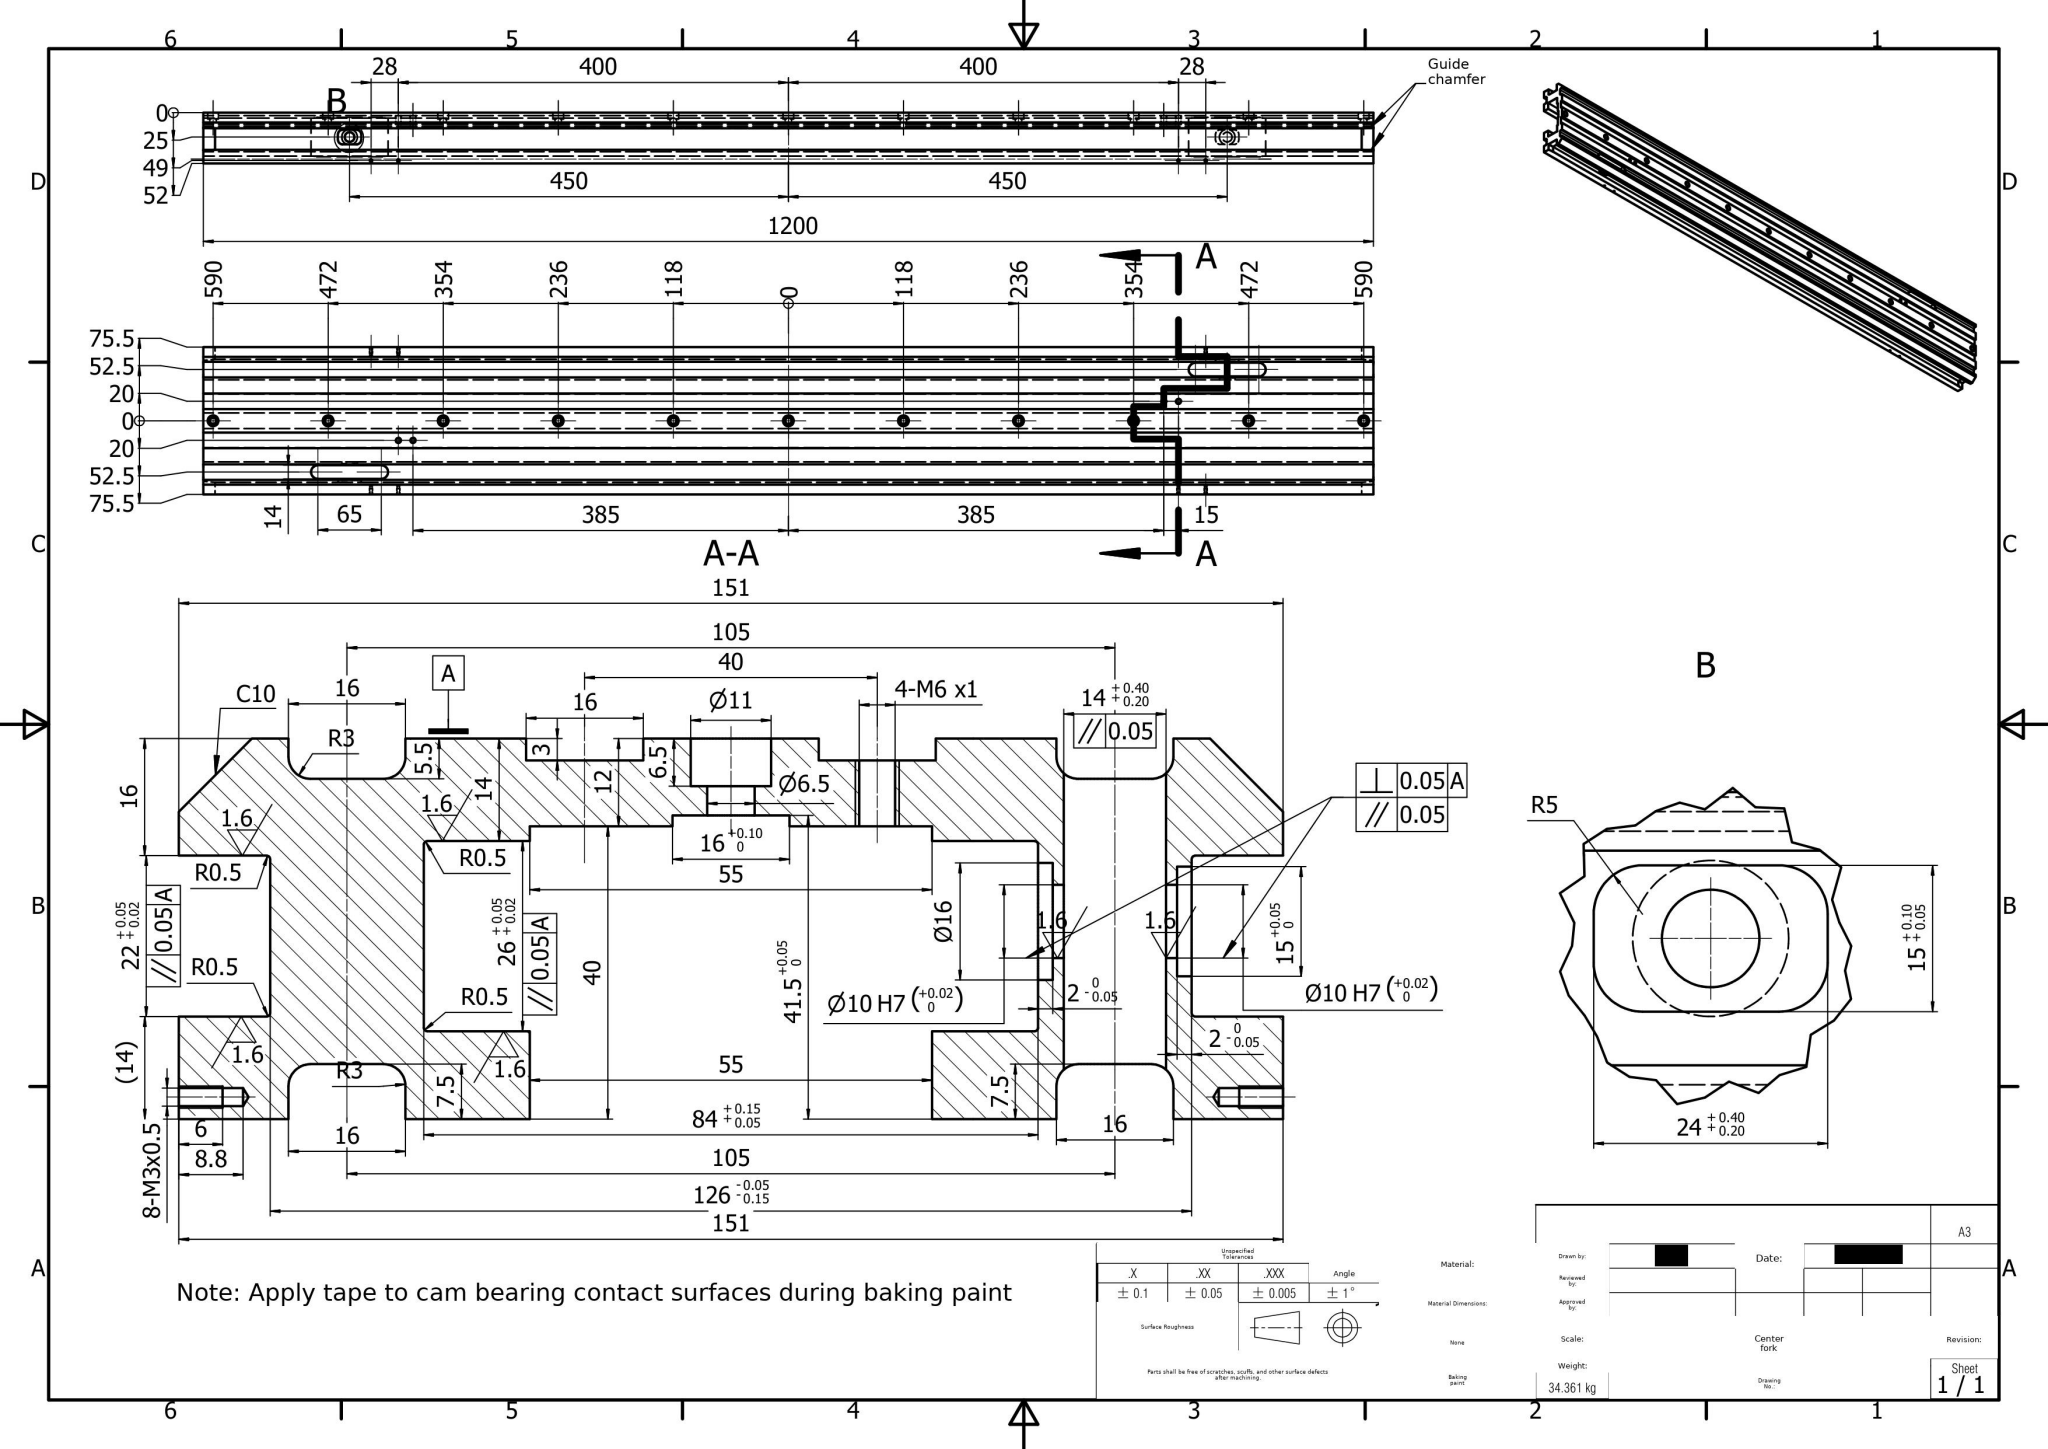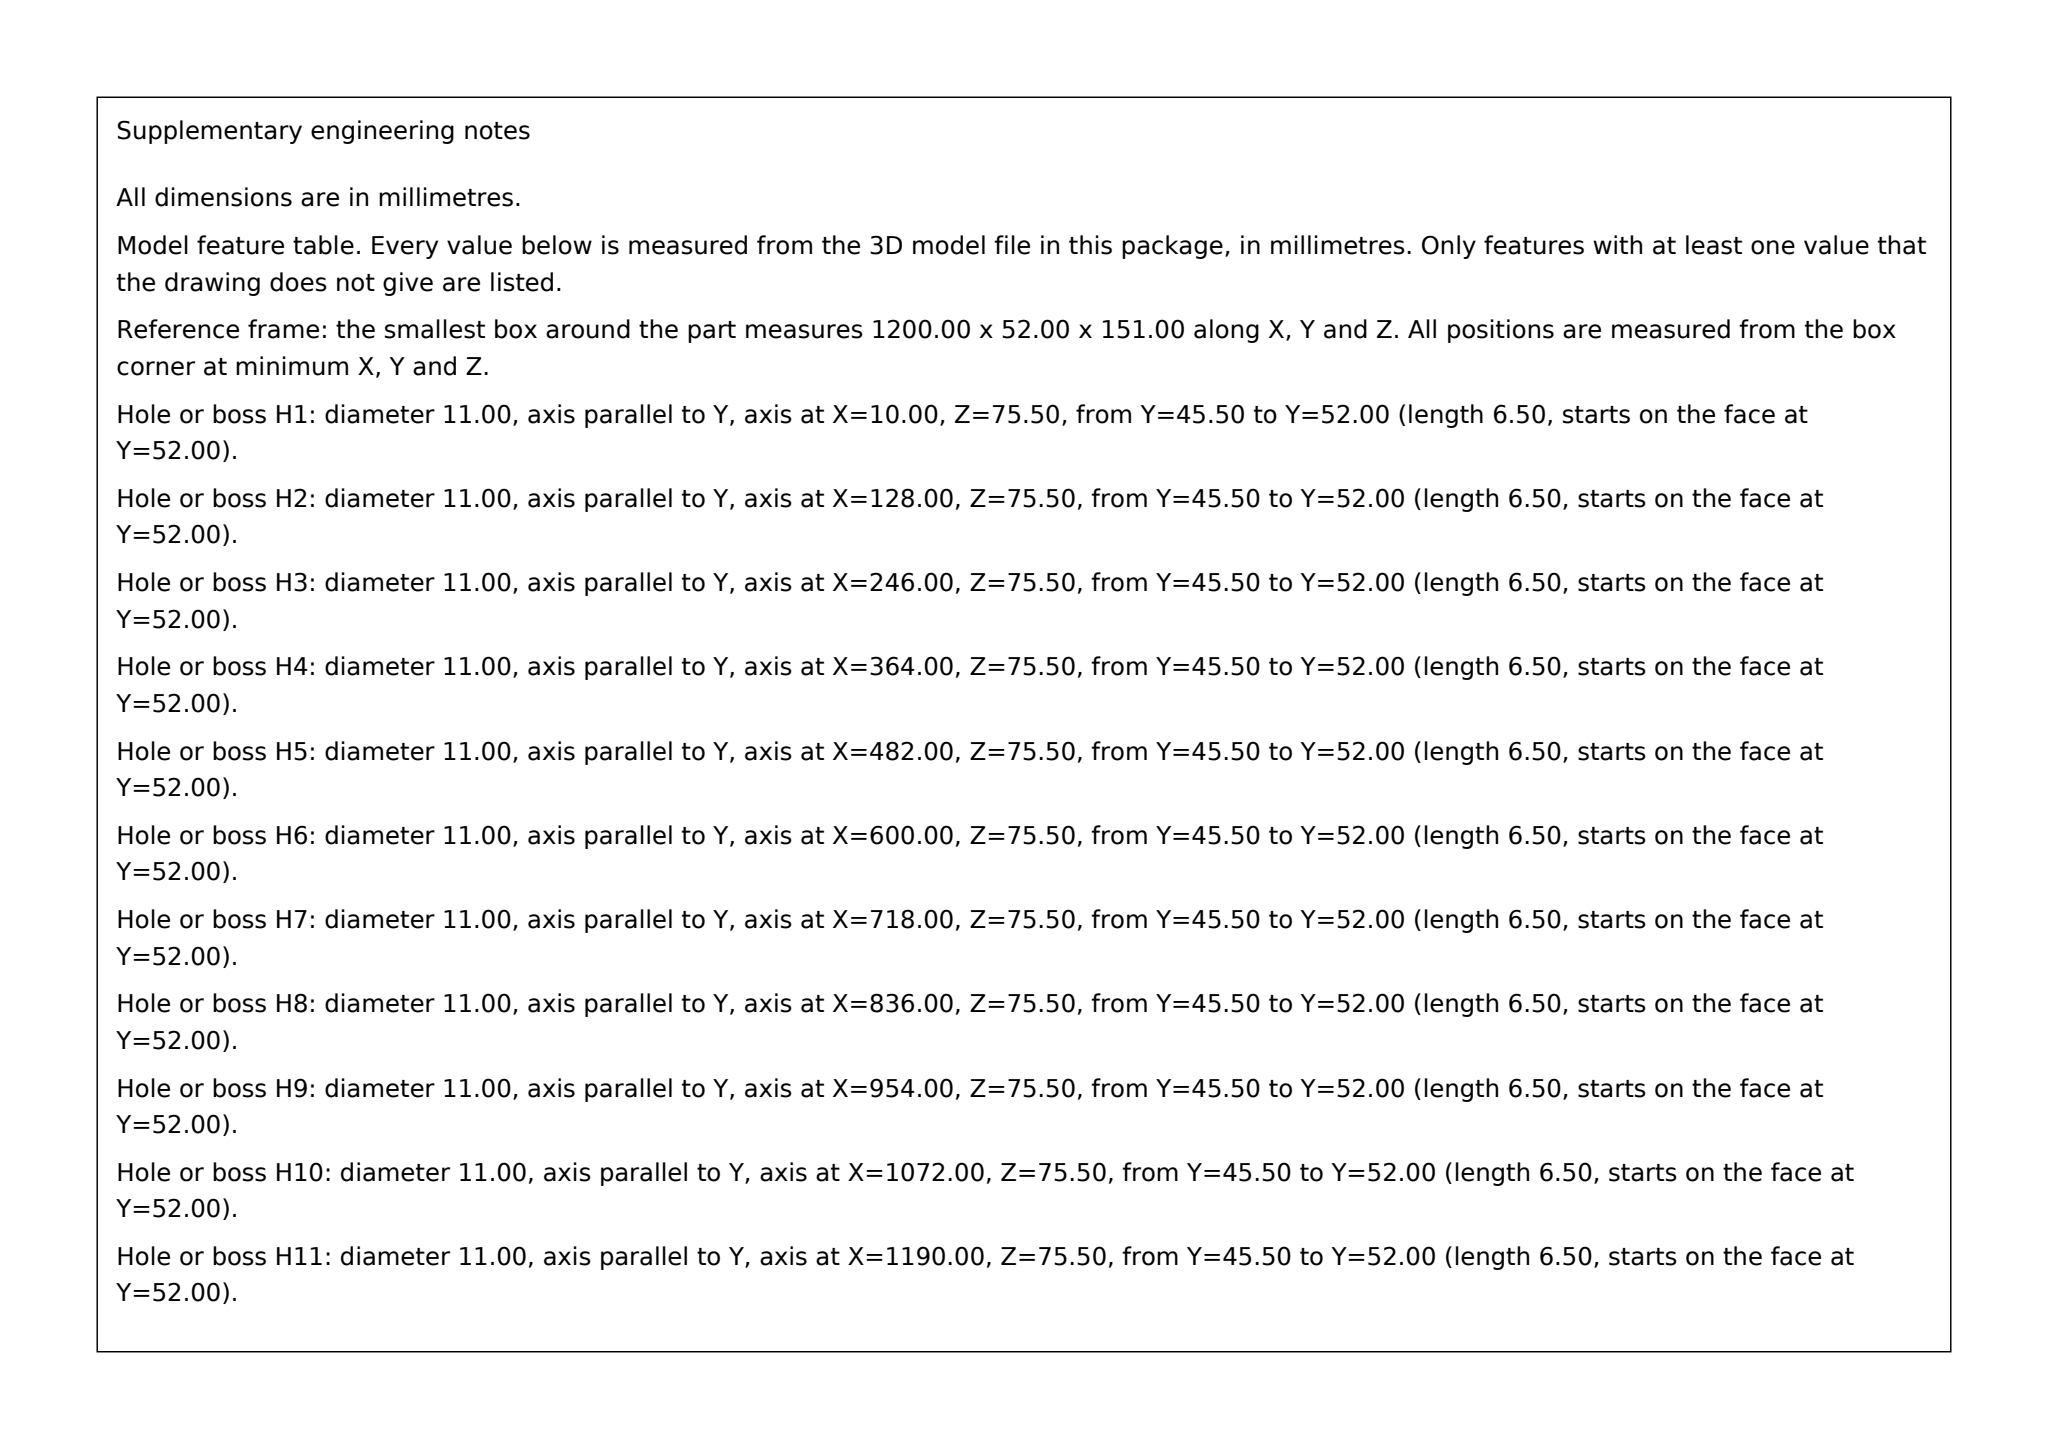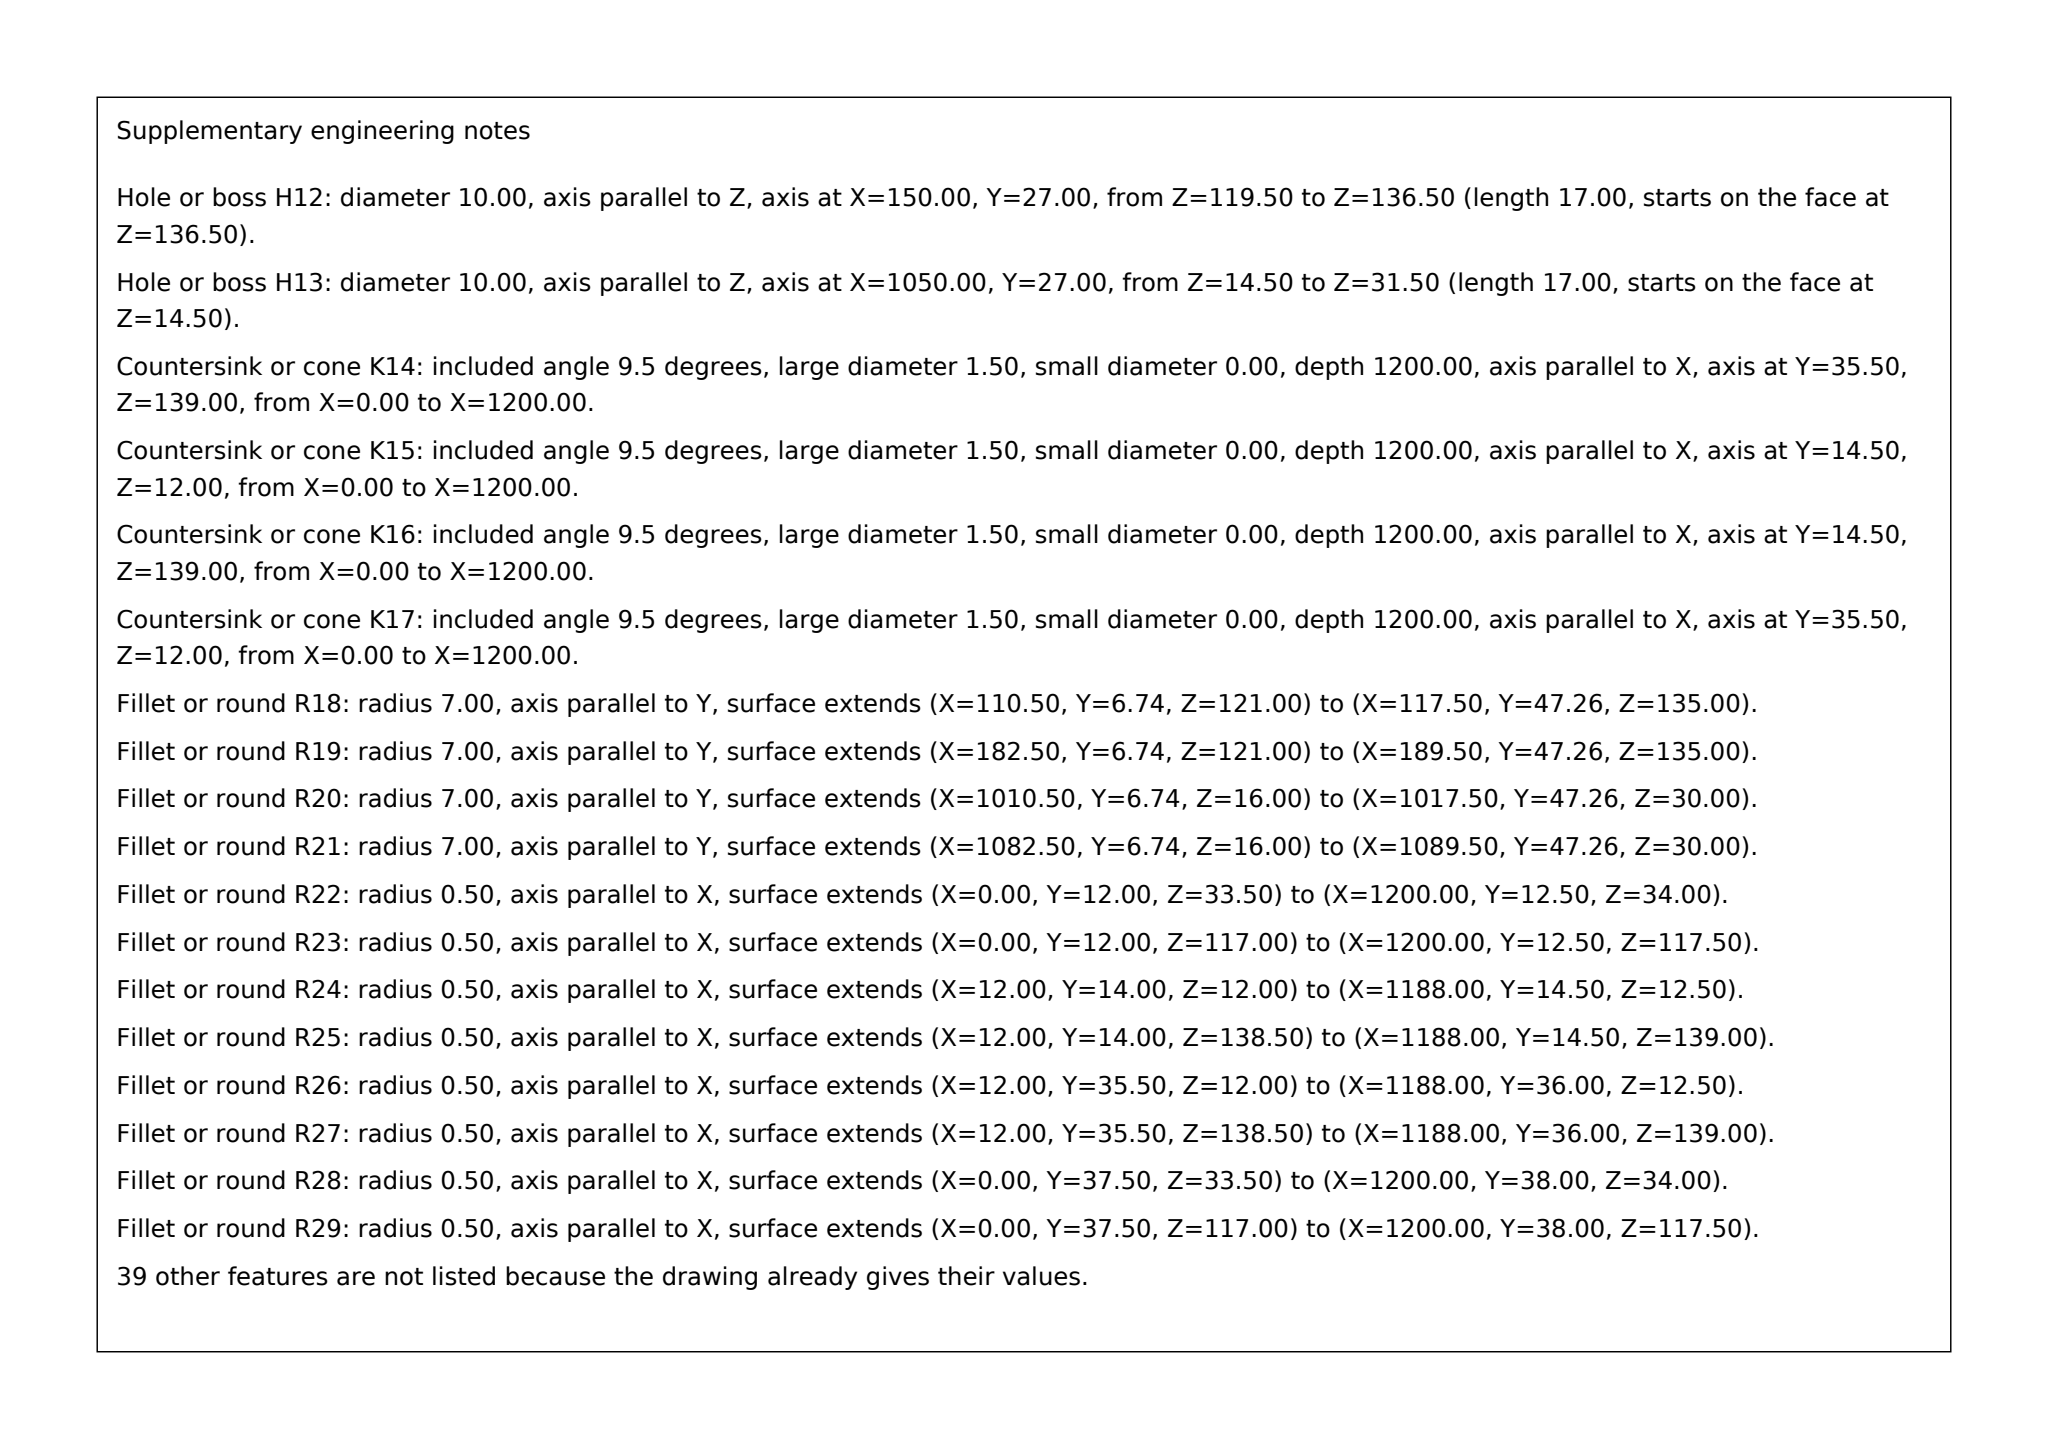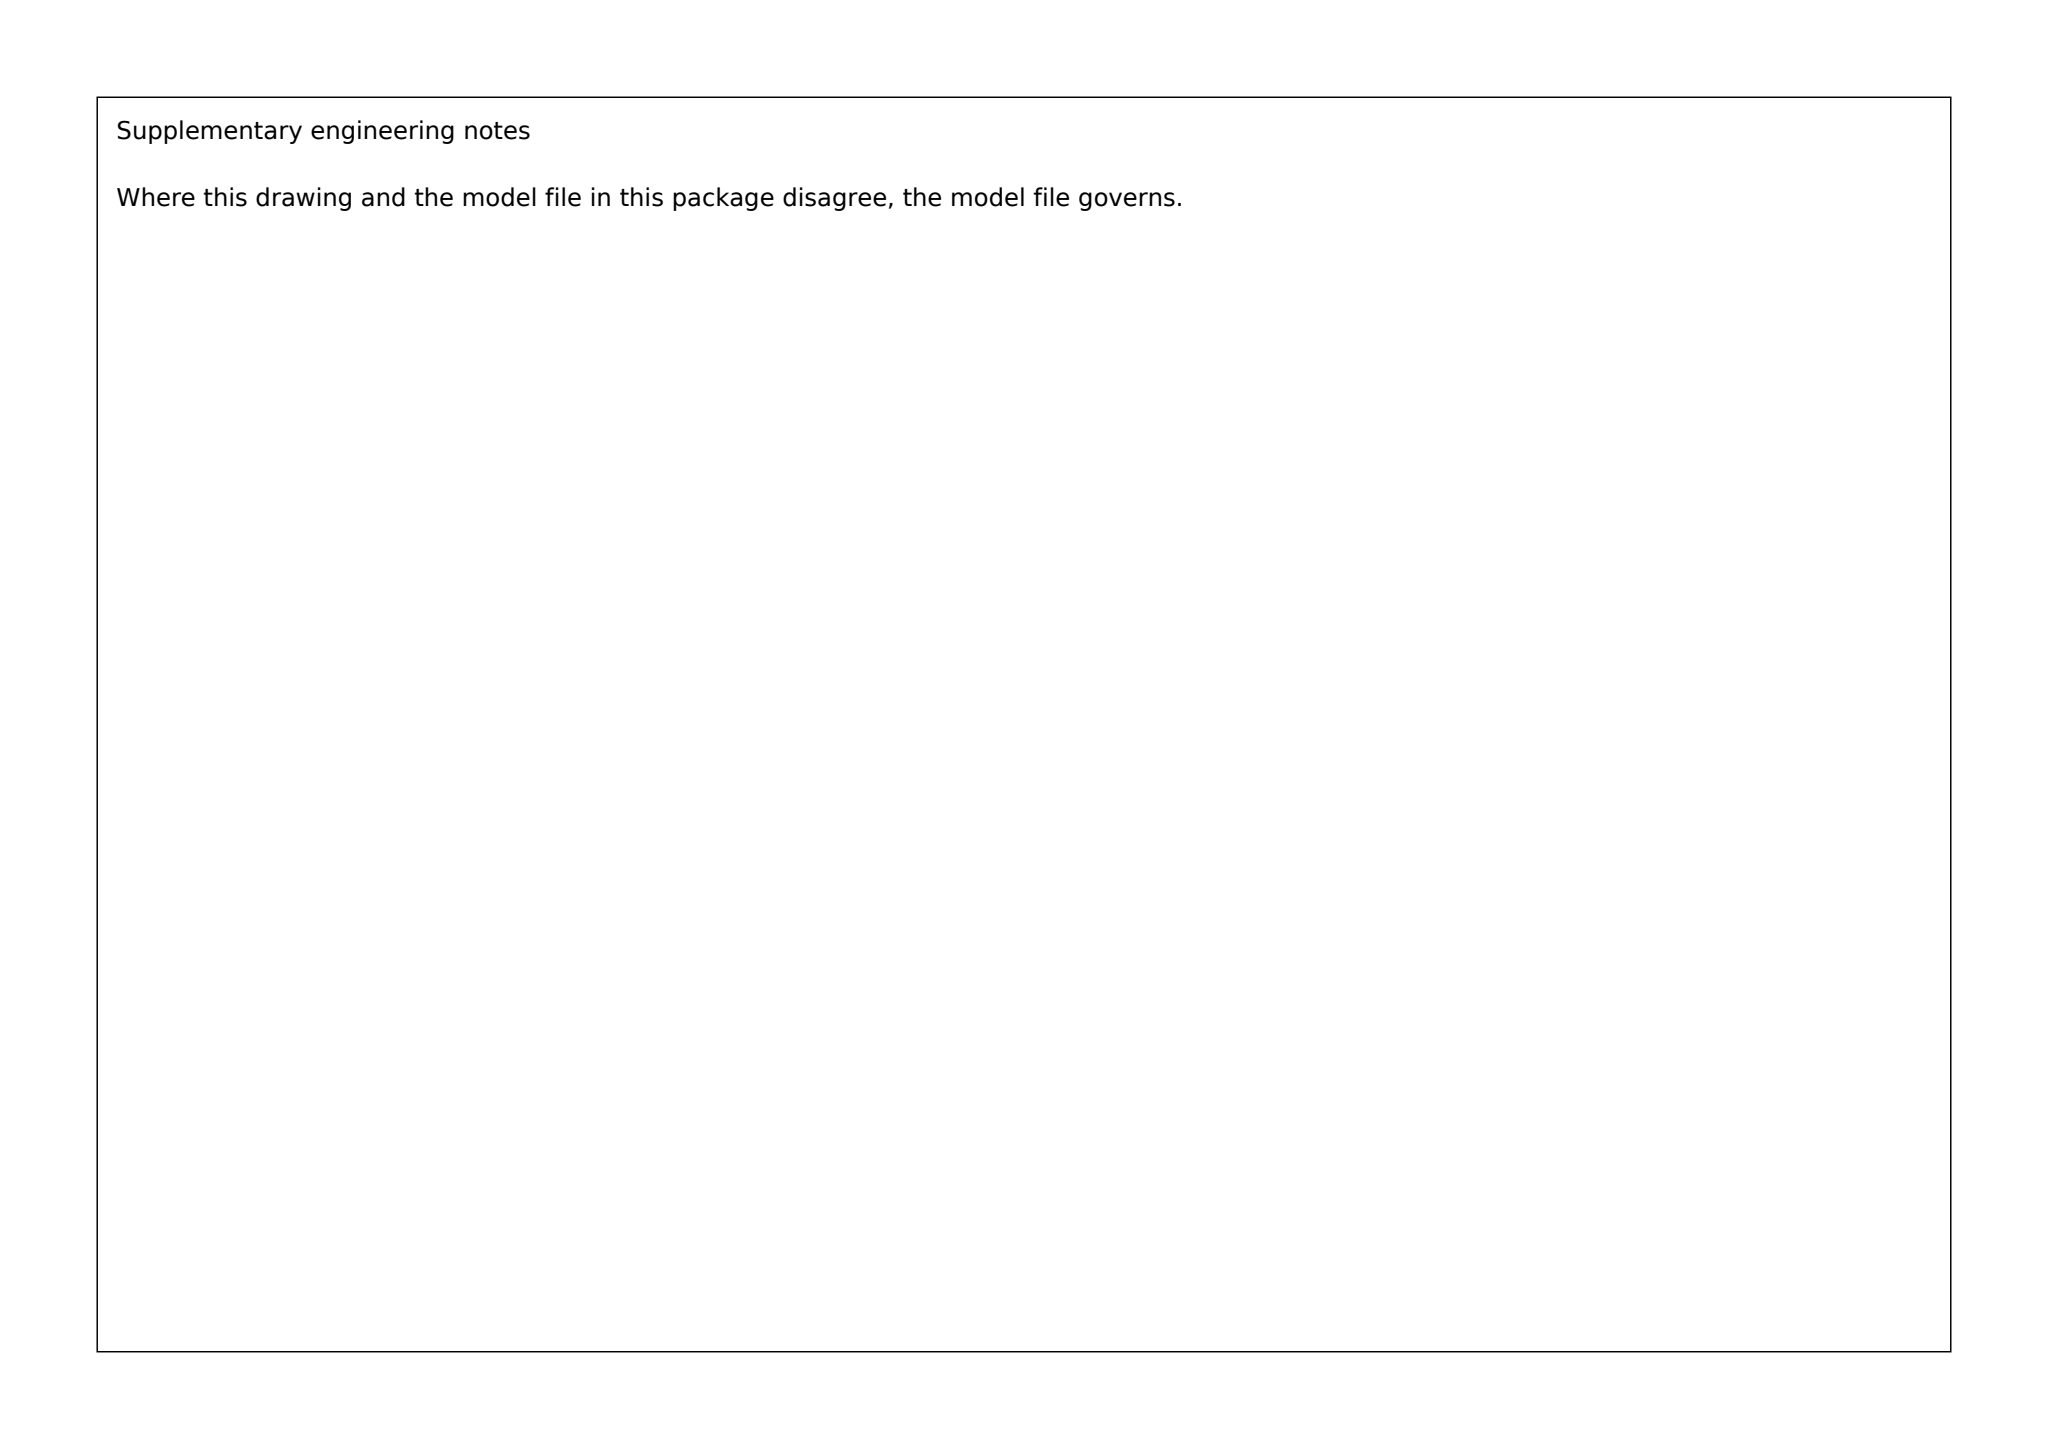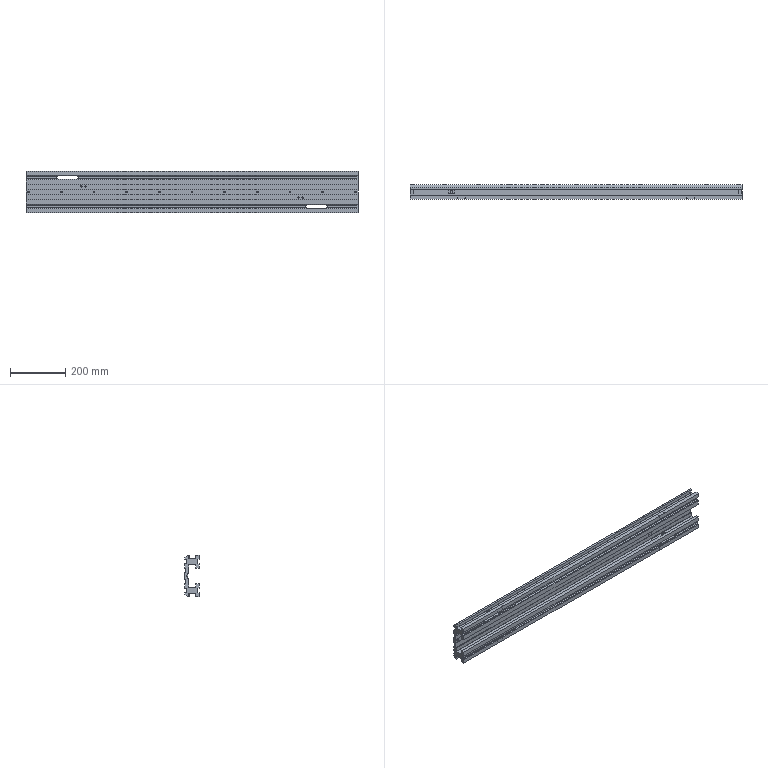Part | SolidWorks | mm | material None | 1 solid | 231 faces | box 1200 x 52 x 151 mm | volume 4377147 mm3 | cylinder 108 | plane 99 | cone 24 | commonest cylinder face diameters 6.5 x22 11 x22 10 x16 2.459 x16 4.917 x8 1 x8 6 x8 16 x4